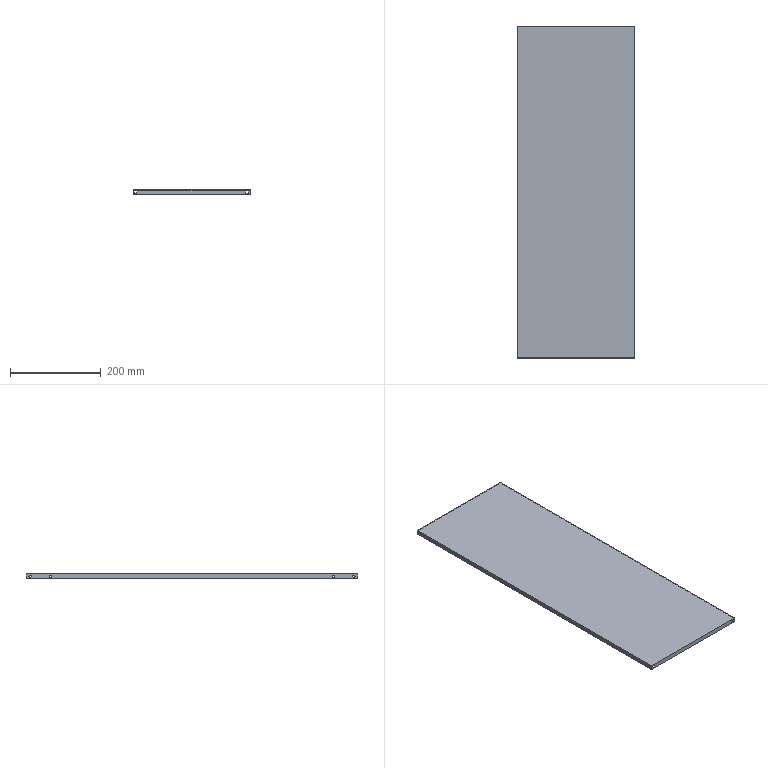Component | SolidWorks | CabinetDoor-2 | 1 solid | 43 faces | box 259 x 732 x 10 mm | volume 309190 mm3 | plane 27 | cylinder 16 | commonest cylinder face diameters 5 x16
build123d program:
from build123d import *

# Parameters (mm, degrees)
SKETCH1_W               = 259
SKETCH1_H               = 732
BOSS_EXTRUDE1_DEPTH     = 10
SHELL1_T                = -1.5
SKETCH2_R               = 2.5
CUT_EXTRUDE1_DEPTH      = 5
SKETCH3_W               = 5
SKETCH3_H               = 5
CUT_EXTRUDE2_DEPTH      = 4
MIRROR2_COPY_1_SKETCH_R = 2.5
MIRROR2_COPY_1_DEPTH    = 5
MIRROR2_COPY_2_SKETCH_W = 5
MIRROR2_COPY_2_SKETCH_H = 5
MIRROR2_COPY_2_DEPTH    = 4


with BuildPart() as part:
    # Sketch1 → Boss-Extrude1 (new body)
    with BuildSketch(Plane.XY):
        with Locations((1.5, 0)):
            Rectangle(SKETCH1_W, SKETCH1_H)
    extrude(amount=BOSS_EXTRUDE1_DEPTH)

    # Shell1
    shell1_openings = [part.faces().sort_by_distance(p)[0] for p in [
        (1.5, 0, 0),
    ]]
    offset(amount=SHELL1_T, openings=shell1_openings, kind=Kind.INTERSECTION)

    # Sketch2 → Cut-Extrude1 (cut)
    with BuildSketch(Plane(origin=(-126.5, 0, 0), x_dir=(0, 0, -1), z_dir=(1, 0, 0))):
        with Locations((-4.25, 357)):
            Circle(SKETCH2_R)
        with Locations((-4.25, 312)):
            Circle(SKETCH2_R)
    cut_extrude1 = extrude(amount=-CUT_EXTRUDE1_DEPTH, mode=Mode.SUBTRACT)

    # Sketch3 → Cut-Extrude2 (cut)
    with BuildSketch(Plane(origin=(0, 366, 0), x_dir=(1, 0, 0), z_dir=(0, 1, 0))):
        with Locations((-123, -5)):
            Rectangle(SKETCH3_W, SKETCH3_H)
    cut_extrude2 = extrude(amount=-CUT_EXTRUDE2_DEPTH, mode=Mode.SUBTRACT)

    # Mirror1: Cut-Extrude1, Cut-Extrude2 across plane
    add(cut_extrude1.mirror(Plane(origin=(0, 0, 0), x_dir=(0, 0, 1), z_dir=(1, 0, 0))), mode=Mode.SUBTRACT)
    add(cut_extrude2.mirror(Plane(origin=(0, 0, 0), x_dir=(0, 0, 1), z_dir=(1, 0, 0))), mode=Mode.SUBTRACT)

    # Mirror2: Cut-Extrude1, Cut-Extrude2 across plane
    add(cut_extrude1.mirror(Plane.ZX), mode=Mode.SUBTRACT)
    add(cut_extrude2.mirror(Plane.ZX), mode=Mode.SUBTRACT)

    # Mirror2 copy 1 sketch → Mirror2 copy 1 (cut)
    with BuildSketch(Plane(origin=(126.5, 0, 0), x_dir=(0, 0, -1), z_dir=(-1, 0, 0))):
        with Locations((-4.25, 357)):
            Circle(MIRROR2_COPY_1_SKETCH_R)
        with Locations((-4.25, 312)):
            Circle(MIRROR2_COPY_1_SKETCH_R)
    extrude(amount=-MIRROR2_COPY_1_DEPTH, mode=Mode.SUBTRACT)

    # Mirror2 copy 2 sketch → Mirror2 copy 2 (cut)
    with BuildSketch(Plane(origin=(0, -366, 0), x_dir=(-1, 0, 0), z_dir=(0, -1, 0))):
        with Locations((-123, -5)):
            Rectangle(MIRROR2_COPY_2_SKETCH_W, MIRROR2_COPY_2_SKETCH_H)
    extrude(amount=-MIRROR2_COPY_2_DEPTH, mode=Mode.SUBTRACT)


solid = part.part

# Placed as in the assembly
solid = solid.moved(Location((129, 400, 290), (0, 0, 0)))